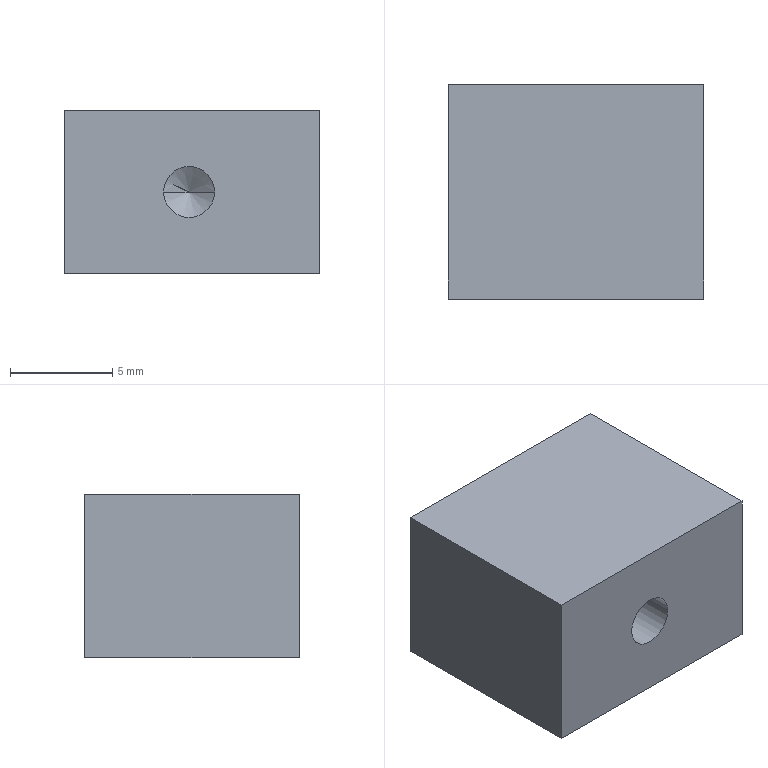CAM job | Mastercam | mm | 8 operations | part box 12.5 x 10.5 x 8
1. Facing | 24 - 100 平铣刀
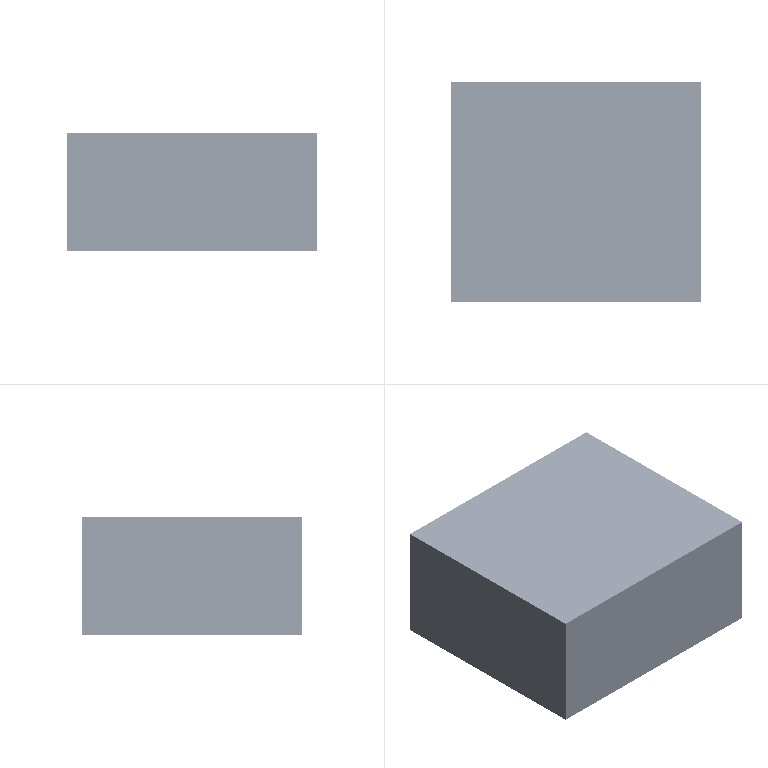2. Contour (Ramp) | 9 - 10 平铣刀
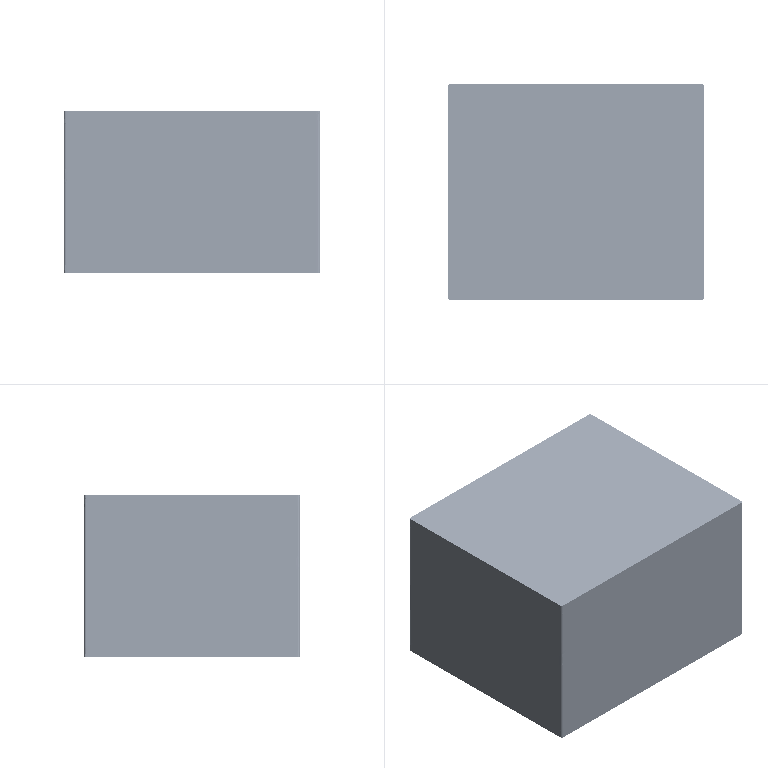3. Contour (2D) | 10 - 10 平铣刀
4. Drill/Counterbore | 5 - 4 倒角刀
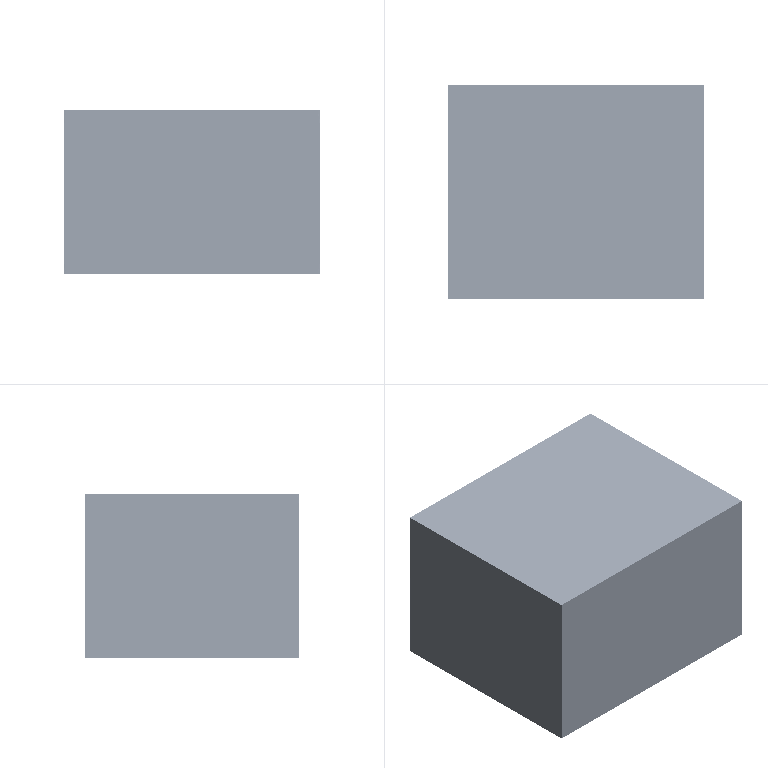5. Contour (2D chamfer) | 5 - 4 倒角刀
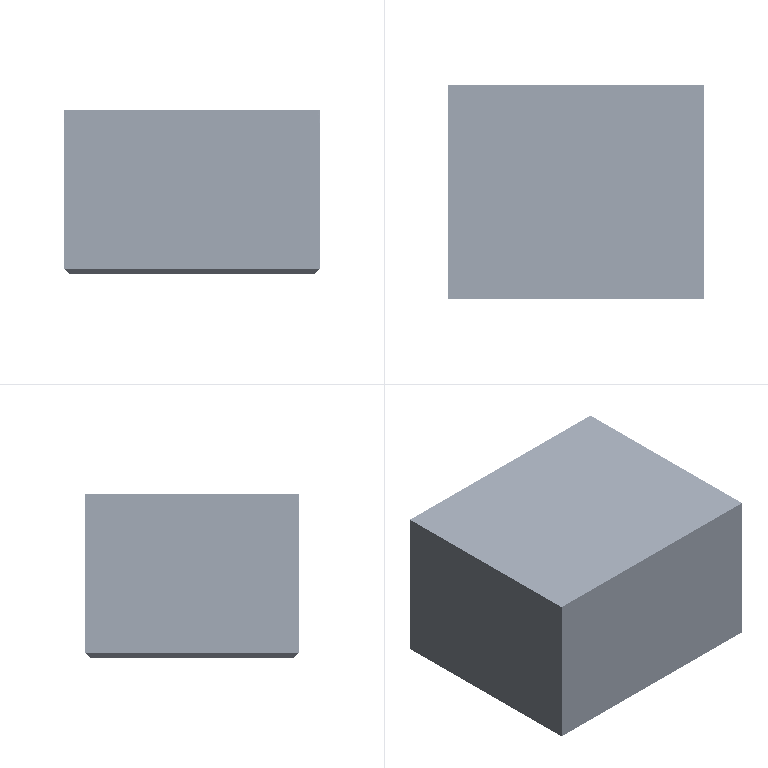6. Facing | 24 - 100 平铣刀
7. Contour (2D chamfer) | 5 - 4 倒角刀
8. Drill/Counterbore | 5 - 4 倒角刀